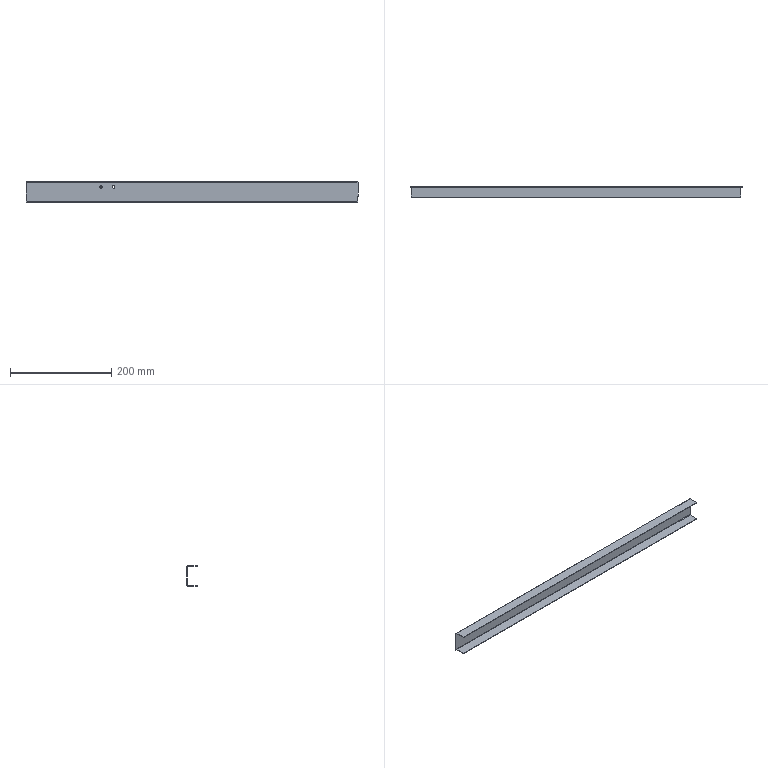Component | SolidWorks | CCQ-1.1-23BendPart-3 | 1 solid | 28 faces | box 655 x 20 x 40 mm | volume 50169 mm3 | plane 20 | cylinder 8 | commonest cylinder face diameters 5 x4 3.473 x2 1.473 x2 | material 304
STEP:
#1=COLOUR_RGB('',0.7922,0.8196,0.9333);
#2=FILL_AREA_STYLE_COLOUR('',#1);
#3=FILL_AREA_STYLE('',(#2));
#4=SURFACE_STYLE_FILL_AREA(#3);
#5=SURFACE_SIDE_STYLE('',(#4));
#6=SURFACE_STYLE_USAGE(.BOTH.,#5);
#7=PRESENTATION_STYLE_ASSIGNMENT((#6));
#8=CARTESIAN_POINT('',(-18.189,-4.114,-3.031));
#9=VERTEX_POINT('',#8);
#10=CARTESIAN_POINT('',(-18.386,-4.114,-3.031));
#11=VERTEX_POINT('',#10);
#12=CARTESIAN_POINT('',(-18.287,-4.114,-3.031));
#13=DIRECTION('',(-0.,1.,0.));
#14=DIRECTION('',(-1.,0.,0.));
#15=AXIS2_PLACEMENT_3D('',#12,#13,#14);
#16=CIRCLE('',#15,0.09843);
#17=EDGE_CURVE('',#9,#11,#16,.T.);
#18=ORIENTED_EDGE('',*,*,#17,.F.);
#19=CARTESIAN_POINT('',(-18.189,-4.075,-3.031));
#20=VERTEX_POINT('',#19);
#21=CARTESIAN_POINT('',(-18.189,-4.469,-3.031));
#22=DIRECTION('',(-0.,1.,0.));
#23=VECTOR('',#22,39.37);
#24=LINE('',#21,#23);
#25=EDGE_CURVE('',#9,#20,#24,.T.);
#26=ORIENTED_EDGE('',*,*,#25,.T.);
#27=CARTESIAN_POINT('',(-18.386,-4.075,-3.031));
#28=VERTEX_POINT('',#27);
#29=CARTESIAN_POINT('',(-18.287,-4.075,-3.031));
#30=DIRECTION('',(-0.,1.,0.));
#31=DIRECTION('',(-1.,0.,0.));
#32=AXIS2_PLACEMENT_3D('',#29,#30,#31);
#33=CIRCLE('',#32,0.09843);
#34=EDGE_CURVE('',#20,#28,#33,.T.);
#35=ORIENTED_EDGE('',*,*,#34,.T.);
#36=CARTESIAN_POINT('',(-18.386,-4.469,-3.031));
#37=DIRECTION('',(-0.,1.,0.));
#38=VECTOR('',#37,39.37);
#39=LINE('',#36,#38);
#40=EDGE_CURVE('',#11,#28,#39,.T.);
#41=ORIENTED_EDGE('',*,*,#40,.F.);
#42=EDGE_LOOP('',(#18,#26,#35,#41));
#43=FACE_OUTER_BOUND('',#42,.T.);
#44=CARTESIAN_POINT('',(-18.287,-4.469,-3.031));
#45=DIRECTION('',(-0.,1.,0.));
#46=DIRECTION('',(-1.,0.,0.));
#47=AXIS2_PLACEMENT_3D('',#44,#45,#46);
#48=CYLINDRICAL_SURFACE('',#47,0.09843);
#49=ADVANCED_FACE('',(#43),#48,.F.);
#50=CARTESIAN_POINT('',(-19.173,-4.114,-3.031));
#51=VERTEX_POINT('',#50);
#52=CARTESIAN_POINT('',(-19.37,-4.114,-3.031));
#53=VERTEX_POINT('',#52);
#54=CARTESIAN_POINT('',(-19.272,-4.114,-3.031));
#55=DIRECTION('',(-0.,1.,0.));
#56=DIRECTION('',(-1.,0.,0.));
#57=AXIS2_PLACEMENT_3D('',#54,#55,#56);
#58=CIRCLE('',#57,0.09843);
#59=EDGE_CURVE('',#51,#53,#58,.T.);
#60=ORIENTED_EDGE('',*,*,#59,.F.);
#61=CARTESIAN_POINT('',(-19.173,-4.075,-3.031));
#62=VERTEX_POINT('',#61);
#63=CARTESIAN_POINT('',(-19.173,-4.469,-3.031));
#64=DIRECTION('',(-0.,1.,0.));
#65=VECTOR('',#64,39.37);
#66=LINE('',#63,#65);
#67=EDGE_CURVE('',#51,#62,#66,.T.);
#68=ORIENTED_EDGE('',*,*,#67,.T.);
#69=CARTESIAN_POINT('',(-19.37,-4.075,-3.031));
#70=VERTEX_POINT('',#69);
#71=CARTESIAN_POINT('',(-19.272,-4.075,-3.031));
#72=DIRECTION('',(-0.,1.,0.));
#73=DIRECTION('',(-1.,0.,0.));
#74=AXIS2_PLACEMENT_3D('',#71,#72,#73);
#75=CIRCLE('',#74,0.09843);
#76=EDGE_CURVE('',#62,#70,#75,.T.);
#77=ORIENTED_EDGE('',*,*,#76,.T.);
#78=CARTESIAN_POINT('',(-19.37,-4.469,-3.031));
#79=DIRECTION('',(-0.,1.,0.));
#80=VECTOR('',#79,39.37);
#81=LINE('',#78,#80);
#82=EDGE_CURVE('',#53,#70,#81,.T.);
#83=ORIENTED_EDGE('',*,*,#82,.F.);
#84=EDGE_LOOP('',(#60,#68,#77,#83));
#85=FACE_OUTER_BOUND('',#84,.T.);
#86=CARTESIAN_POINT('',(-19.272,-4.469,-3.031));
#87=DIRECTION('',(-0.,1.,0.));
#88=DIRECTION('',(-1.,0.,0.));
#89=AXIS2_PLACEMENT_3D('',#86,#87,#88);
#90=CYLINDRICAL_SURFACE('',#89,0.09843);
#91=ADVANCED_FACE('',(#85),#90,.F.);
#92=CARTESIAN_POINT('',(-25.098,-4.114,-3.74));
#93=VERTEX_POINT('',#92);
#94=CARTESIAN_POINT('',(-25.098,-4.075,-3.74));
#95=VERTEX_POINT('',#94);
#96=CARTESIAN_POINT('',(-25.098,-4.143,-3.74));
#97=DIRECTION('',(-0.,1.,0.));
#98=VECTOR('',#97,39.37);
#99=LINE('',#96,#98);
#100=EDGE_CURVE('',#93,#95,#99,.T.);
#101=ORIENTED_EDGE('',*,*,#100,.F.);
#102=CARTESIAN_POINT('',(-25.098,-4.114,-2.706));
#103=VERTEX_POINT('',#102);
#104=CARTESIAN_POINT('',(-25.098,-4.114,-4.213));
#105=DIRECTION('',(-0.,-0.,1.));
#106=VECTOR('',#105,39.37);
#107=LINE('',#104,#106);
#108=EDGE_CURVE('',#93,#103,#107,.T.);
#109=ORIENTED_EDGE('',*,*,#108,.T.);
#110=CARTESIAN_POINT('',(-25.098,-4.075,-2.706));
#111=VERTEX_POINT('',#110);
#112=CARTESIAN_POINT('',(-25.098,-4.114,-2.706));
#113=DIRECTION('',(-0.,1.,0.));
#114=VECTOR('',#113,39.37);
#115=LINE('',#112,#114);
#116=EDGE_CURVE('',#103,#111,#115,.T.);
#117=ORIENTED_EDGE('',*,*,#116,.T.);
#118=CARTESIAN_POINT('',(-25.098,-4.075,-4.213));
#119=DIRECTION('',(-0.,-0.,1.));
#120=VECTOR('',#119,39.37);
#121=LINE('',#118,#120);
#122=EDGE_CURVE('',#95,#111,#121,.T.);
#123=ORIENTED_EDGE('',*,*,#122,.F.);
#124=EDGE_LOOP('',(#101,#109,#117,#123));
#125=FACE_OUTER_BOUND('',#124,.T.);
#126=CARTESIAN_POINT('',(-25.098,-4.143,-4.173));
#127=DIRECTION('',(-1.,-0.,-0.));
#128=DIRECTION('',(-0.,-0.,1.));
#129=AXIS2_PLACEMENT_3D('',#126,#127,#128);
#130=PLANE('',#129);
#131=ADVANCED_FACE('',(#125),#130,.T.);
#132=CARTESIAN_POINT('',(-25.098,-4.114,-2.644));
#133=VERTEX_POINT('',#132);
#134=CARTESIAN_POINT('',(-25.098,-4.114,-2.638));
#135=DIRECTION('',(0.,0.,-1.));
#136=VECTOR('',#135,39.37);
#137=LINE('',#134,#136);
#138=EDGE_CURVE('',#133,#103,#137,.T.);
#139=ORIENTED_EDGE('',*,*,#138,.F.);
#140=CARTESIAN_POINT('',(-25.098,-4.143,-2.706));
#141=DIRECTION('',(1.,0.,0.));
#142=DIRECTION('',(0.,0.,1.));
#143=AXIS2_PLACEMENT_3D('',#140,#141,#142);
#144=CIRCLE('',#143,0.06837);
#145=EDGE_CURVE('',#111,#133,#144,.T.);
#146=ORIENTED_EDGE('',*,*,#145,.F.);
#147=ORIENTED_EDGE('',*,*,#116,.F.);
#148=EDGE_LOOP('',(#139,#146,#147));
#149=FACE_OUTER_BOUND('',#148,.T.);
#150=CARTESIAN_POINT('',(-25.098,-4.143,-2.638));
#151=DIRECTION('',(-1.,-0.,-0.));
#152=DIRECTION('',(-0.,-0.,1.));
#153=AXIS2_PLACEMENT_3D('',#150,#151,#152);
#154=PLANE('',#153);
#155=ADVANCED_FACE('',(#149),#154,.T.);
#156=CARTESIAN_POINT('',(0.689,-4.114,-2.706));
#157=VERTEX_POINT('',#156);
#158=CARTESIAN_POINT('',(0.689,-4.114,-2.644));
#159=VERTEX_POINT('',#158);
#160=CARTESIAN_POINT('',(0.689,-4.114,-2.706));
#161=DIRECTION('',(-0.,-0.,1.));
#162=VECTOR('',#161,39.37);
#163=LINE('',#160,#162);
#164=EDGE_CURVE('',#157,#159,#163,.T.);
#165=ORIENTED_EDGE('',*,*,#164,.F.);
#166=CARTESIAN_POINT('',(0.689,-4.075,-2.706));
#167=VERTEX_POINT('',#166);
#168=CARTESIAN_POINT('',(0.689,-4.075,-2.706));
#169=DIRECTION('',(0.,-1.,-0.));
#170=VECTOR('',#169,39.37);
#171=LINE('',#168,#170);
#172=EDGE_CURVE('',#167,#157,#171,.T.);
#173=ORIENTED_EDGE('',*,*,#172,.F.);
#174=CARTESIAN_POINT('',(0.689,-4.143,-2.706));
#175=DIRECTION('',(1.,0.,0.));
#176=DIRECTION('',(0.,0.,1.));
#177=AXIS2_PLACEMENT_3D('',#174,#175,#176);
#178=CIRCLE('',#177,0.06837);
#179=EDGE_CURVE('',#167,#159,#178,.T.);
#180=ORIENTED_EDGE('',*,*,#179,.T.);
#181=EDGE_LOOP('',(#165,#173,#180));
#182=FACE_OUTER_BOUND('',#181,.T.);
#183=CARTESIAN_POINT('',(0.689,-4.075,-2.706));
#184=DIRECTION('',(1.,0.,0.));
#185=DIRECTION('',(0.,0.,-1.));
#186=AXIS2_PLACEMENT_3D('',#183,#184,#185);
#187=PLANE('',#186);
#188=ADVANCED_FACE('',(#182),#187,.T.);
#189=CARTESIAN_POINT('',(0.689,-4.075,-3.74));
#190=VERTEX_POINT('',#189);
#191=CARTESIAN_POINT('',(0.689,-4.114,-3.74));
#192=VERTEX_POINT('',#191);
#193=CARTESIAN_POINT('',(0.689,-4.143,-3.74));
#194=DIRECTION('',(0.,-1.,-0.));
#195=VECTOR('',#194,39.37);
#196=LINE('',#193,#195);
#197=EDGE_CURVE('',#190,#192,#196,.T.);
#198=ORIENTED_EDGE('',*,*,#197,.F.);
#199=CARTESIAN_POINT('',(0.689,-4.075,-4.213));
#200=DIRECTION('',(-0.,-0.,1.));
#201=VECTOR('',#200,39.37);
#202=LINE('',#199,#201);
#203=EDGE_CURVE('',#190,#167,#202,.T.);
#204=ORIENTED_EDGE('',*,*,#203,.T.);
#205=ORIENTED_EDGE('',*,*,#172,.T.);
#206=CARTESIAN_POINT('',(0.689,-4.114,-4.213));
#207=DIRECTION('',(-0.,-0.,1.));
#208=VECTOR('',#207,39.37);
#209=LINE('',#206,#208);
#210=EDGE_CURVE('',#192,#157,#209,.T.);
#211=ORIENTED_EDGE('',*,*,#210,.F.);
#212=EDGE_LOOP('',(#198,#204,#205,#211));
#213=FACE_OUTER_BOUND('',#212,.T.);
#214=CARTESIAN_POINT('',(0.689,-4.143,-2.677));
#215=DIRECTION('',(1.,0.,0.));
#216=DIRECTION('',(0.,0.,-1.));
#217=AXIS2_PLACEMENT_3D('',#214,#215,#216);
#218=PLANE('',#217);
#219=ADVANCED_FACE('',(#213),#218,.T.);
#220=CARTESIAN_POINT('',(-25.008,-4.862,-2.677));
#221=VERTEX_POINT('',#220);
#222=CARTESIAN_POINT('',(0.5984,-4.862,-2.677));
#223=VERTEX_POINT('',#222);
#224=CARTESIAN_POINT('',(-25.098,-4.862,-2.677));
#225=DIRECTION('',(1.,0.,0.));
#226=VECTOR('',#225,39.37);
#227=LINE('',#224,#226);
#228=EDGE_CURVE('',#221,#223,#227,.T.);
#229=ORIENTED_EDGE('',*,*,#228,.F.);
#230=CARTESIAN_POINT('',(-25.008,-4.143,-2.677));
#231=VERTEX_POINT('',#230);
#232=CARTESIAN_POINT('',(-25.008,-4.075,-2.677));
#233=DIRECTION('',(-0.,1.,0.));
#234=VECTOR('',#233,39.37);
#235=LINE('',#232,#234);
#236=EDGE_CURVE('',#221,#231,#235,.T.);
#237=ORIENTED_EDGE('',*,*,#236,.T.);
#238=CARTESIAN_POINT('',(0.5984,-4.143,-2.677));
#239=VERTEX_POINT('',#238);
#240=CARTESIAN_POINT('',(-25.098,-4.143,-2.677));
#241=DIRECTION('',(1.,0.,0.));
#242=VECTOR('',#241,39.37);
#243=LINE('',#240,#242);
#244=EDGE_CURVE('',#231,#239,#243,.T.);
#245=ORIENTED_EDGE('',*,*,#244,.T.);
#246=CARTESIAN_POINT('',(0.5984,-4.075,-2.677));
#247=DIRECTION('',(0.,-1.,-0.));
#248=VECTOR('',#247,39.37);
#249=LINE('',#246,#248);
#250=EDGE_CURVE('',#239,#223,#249,.T.);
#251=ORIENTED_EDGE('',*,*,#250,.T.);
#252=EDGE_LOOP('',(#229,#237,#245,#251));
#253=FACE_OUTER_BOUND('',#252,.T.);
#254=CARTESIAN_POINT('',(-25.098,-4.075,-2.677));
#255=DIRECTION('',(-0.,-0.,1.));
#256=DIRECTION('',(-0.,1.,0.));
#257=AXIS2_PLACEMENT_3D('',#254,#255,#256);
#258=PLANE('',#257);
#259=ADVANCED_FACE('',(#253),#258,.F.);
#260=CARTESIAN_POINT('',(-25.008,-4.862,-2.638));
#261=VERTEX_POINT('',#260);
#262=CARTESIAN_POINT('',(-25.008,-4.862,-2.638));
#263=DIRECTION('',(-0.,-0.,1.));
#264=VECTOR('',#263,39.37);
#265=LINE('',#262,#264);
#266=EDGE_CURVE('',#221,#261,#265,.T.);
#267=ORIENTED_EDGE('',*,*,#266,.F.);
#268=ORIENTED_EDGE('',*,*,#228,.T.);
#269=CARTESIAN_POINT('',(0.5984,-4.862,-2.638));
#270=VERTEX_POINT('',#269);
#271=CARTESIAN_POINT('',(0.5984,-4.862,-2.638));
#272=DIRECTION('',(0.,0.,-1.));
#273=VECTOR('',#272,39.37);
#274=LINE('',#271,#273);
#275=EDGE_CURVE('',#270,#223,#274,.T.);
#276=ORIENTED_EDGE('',*,*,#275,.F.);
#277=CARTESIAN_POINT('',(-25.098,-4.862,-2.638));
#278=DIRECTION('',(1.,0.,0.));
#279=VECTOR('',#278,39.37);
#280=LINE('',#277,#279);
#281=EDGE_CURVE('',#261,#270,#280,.T.);
#282=ORIENTED_EDGE('',*,*,#281,.F.);
#283=EDGE_LOOP('',(#267,#268,#276,#282));
#284=FACE_OUTER_BOUND('',#283,.T.);
#285=CARTESIAN_POINT('',(-25.098,-4.862,-2.638));
#286=DIRECTION('',(0.,-1.,-0.));
#287=DIRECTION('',(1.,0.,0.));
#288=AXIS2_PLACEMENT_3D('',#285,#286,#287);
#289=PLANE('',#288);
#290=ADVANCED_FACE('',(#284),#289,.T.);
#291=CARTESIAN_POINT('',(-25.008,-4.143,-2.638));
#292=VERTEX_POINT('',#291);
#293=CARTESIAN_POINT('',(-25.008,-4.075,-2.638));
#294=DIRECTION('',(-0.,1.,0.));
#295=VECTOR('',#294,39.37);
#296=LINE('',#293,#295);
#297=EDGE_CURVE('',#261,#292,#296,.T.);
#298=ORIENTED_EDGE('',*,*,#297,.F.);
#299=ORIENTED_EDGE('',*,*,#281,.T.);
#300=CARTESIAN_POINT('',(0.5984,-4.143,-2.638));
#301=VERTEX_POINT('',#300);
#302=CARTESIAN_POINT('',(0.5984,-4.075,-2.638));
#303=DIRECTION('',(0.,-1.,-0.));
#304=VECTOR('',#303,39.37);
#305=LINE('',#302,#304);
#306=EDGE_CURVE('',#301,#270,#305,.T.);
#307=ORIENTED_EDGE('',*,*,#306,.F.);
#308=CARTESIAN_POINT('',(-25.098,-4.143,-2.638));
#309=DIRECTION('',(1.,0.,0.));
#310=VECTOR('',#309,39.37);
#311=LINE('',#308,#310);
#312=EDGE_CURVE('',#292,#301,#311,.T.);
#313=ORIENTED_EDGE('',*,*,#312,.F.);
#314=EDGE_LOOP('',(#298,#299,#307,#313));
#315=FACE_OUTER_BOUND('',#314,.T.);
#316=CARTESIAN_POINT('',(-25.098,-4.075,-2.638));
#317=DIRECTION('',(-0.,-0.,1.));
#318=DIRECTION('',(-0.,1.,0.));
#319=AXIS2_PLACEMENT_3D('',#316,#317,#318);
#320=PLANE('',#319);
#321=ADVANCED_FACE('',(#315),#320,.T.);
#322=CARTESIAN_POINT('',(-25.008,-4.114,-2.644));
#323=VERTEX_POINT('',#322);
#324=CARTESIAN_POINT('',(-25.098,-4.114,-2.644));
#325=DIRECTION('',(-1.,-0.,-0.));
#326=VECTOR('',#325,39.37);
#327=LINE('',#324,#326);
#328=EDGE_CURVE('',#323,#133,#327,.T.);
#329=ORIENTED_EDGE('',*,*,#328,.F.);
#330=CARTESIAN_POINT('',(-25.008,-4.143,-2.706));
#331=DIRECTION('',(-1.,-0.,-0.));
#332=DIRECTION('',(0.,-0.,-1.));
#333=AXIS2_PLACEMENT_3D('',#330,#331,#332);
#334=CIRCLE('',#333,0.06837);
#335=EDGE_CURVE('',#292,#323,#334,.T.);
#336=ORIENTED_EDGE('',*,*,#335,.F.);
#337=ORIENTED_EDGE('',*,*,#312,.T.);
#338=CARTESIAN_POINT('',(0.5984,-4.114,-2.644));
#339=VERTEX_POINT('',#338);
#340=CARTESIAN_POINT('',(0.5984,-4.143,-2.706));
#341=DIRECTION('',(1.,0.,0.));
#342=DIRECTION('',(0.,-0.,1.));
#343=AXIS2_PLACEMENT_3D('',#340,#341,#342);
#344=CIRCLE('',#343,0.06837);
#345=EDGE_CURVE('',#339,#301,#344,.T.);
#346=ORIENTED_EDGE('',*,*,#345,.F.);
#347=CARTESIAN_POINT('',(-25.098,-4.114,-2.644));
#348=DIRECTION('',(-1.,-0.,-0.));
#349=VECTOR('',#348,39.37);
#350=LINE('',#347,#349);
#351=EDGE_CURVE('',#159,#339,#350,.T.);
#352=ORIENTED_EDGE('',*,*,#351,.F.);
#353=ORIENTED_EDGE('',*,*,#179,.F.);
#354=CARTESIAN_POINT('',(-25.098,-4.075,-2.706));
#355=DIRECTION('',(1.,0.,0.));
#356=VECTOR('',#355,39.37);
#357=LINE('',#354,#356);
#358=EDGE_CURVE('',#111,#167,#357,.T.);
#359=ORIENTED_EDGE('',*,*,#358,.F.);
#360=ORIENTED_EDGE('',*,*,#145,.T.);
#361=EDGE_LOOP('',(#329,#336,#337,#346,#352,#353,#359,#360));
#362=FACE_OUTER_BOUND('',#361,.T.);
#363=CARTESIAN_POINT('',(-25.098,-4.143,-2.706));
#364=DIRECTION('',(1.,0.,0.));
#365=DIRECTION('',(0.,0.,-1.));
#366=AXIS2_PLACEMENT_3D('',#363,#364,#365);
#367=CYLINDRICAL_SURFACE('',#366,0.06837);
#368=ADVANCED_FACE('',(#362),#367,.T.);
#369=CARTESIAN_POINT('',(-25.079,-4.075,-3.74));
#370=VERTEX_POINT('',#369);
#371=CARTESIAN_POINT('',(-25.079,-4.075,-4.144));
#372=VERTEX_POINT('',#371);
#373=CARTESIAN_POINT('',(-25.079,-4.075,-4.213));
#374=DIRECTION('',(0.,0.,-1.));
#375=VECTOR('',#374,39.37);
#376=LINE('',#373,#375);
#377=EDGE_CURVE('',#370,#372,#376,.T.);
#378=ORIENTED_EDGE('',*,*,#377,.F.);
#379=CARTESIAN_POINT('',(-25.098,-4.075,-3.74));
#380=DIRECTION('',(1.,0.,0.));
#381=VECTOR('',#380,39.37);
#382=LINE('',#379,#381);
#383=EDGE_CURVE('',#95,#370,#382,.T.);
#384=ORIENTED_EDGE('',*,*,#383,.F.);
#385=ORIENTED_EDGE('',*,*,#122,.T.);
#386=ORIENTED_EDGE('',*,*,#358,.T.);
#387=ORIENTED_EDGE('',*,*,#203,.F.);
#388=CARTESIAN_POINT('',(0.6693,-4.075,-3.74));
#389=VERTEX_POINT('',#388);
#390=CARTESIAN_POINT('',(-25.098,-4.075,-3.74));
#391=DIRECTION('',(1.,0.,0.));
#392=VECTOR('',#391,39.37);
#393=LINE('',#390,#392);
#394=EDGE_CURVE('',#389,#190,#393,.T.);
#395=ORIENTED_EDGE('',*,*,#394,.F.);
#396=CARTESIAN_POINT('',(0.6693,-4.075,-4.144));
#397=VERTEX_POINT('',#396);
#398=CARTESIAN_POINT('',(0.6693,-4.075,-4.213));
#399=DIRECTION('',(-0.,-0.,1.));
#400=VECTOR('',#399,39.37);
#401=LINE('',#398,#400);
#402=EDGE_CURVE('',#397,#389,#401,.T.);
#403=ORIENTED_EDGE('',*,*,#402,.F.);
#404=CARTESIAN_POINT('',(-25.098,-4.075,-4.144));
#405=DIRECTION('',(1.,0.,0.));
#406=VECTOR('',#405,39.37);
#407=LINE('',#404,#406);
#408=EDGE_CURVE('',#372,#397,#407,.T.);
#409=ORIENTED_EDGE('',*,*,#408,.F.);
#410=EDGE_LOOP('',(#378,#384,#385,#386,#387,#395,#403,#409));
#411=FACE_OUTER_BOUND('',#410,.T.);
#412=CARTESIAN_POINT('',(-18.287,-4.075,-3.031));
#413=DIRECTION('',(-0.,1.,0.));
#414=DIRECTION('',(-1.,0.,0.));
#415=AXIS2_PLACEMENT_3D('',#412,#413,#414);
#416=CIRCLE('',#415,0.09843);
#417=EDGE_CURVE('',#28,#20,#416,.T.);
#418=ORIENTED_EDGE('',*,*,#417,.F.);
#419=ORIENTED_EDGE('',*,*,#34,.F.);
#420=EDGE_LOOP('',(#418,#419));
#421=FACE_BOUND('',#420,.T.);
#422=CARTESIAN_POINT('',(-19.272,-4.075,-3.031));
#423=DIRECTION('',(-0.,1.,0.));
#424=DIRECTION('',(-1.,0.,0.));
#425=AXIS2_PLACEMENT_3D('',#422,#423,#424);
#426=CIRCLE('',#425,0.09843);
#427=EDGE_CURVE('',#70,#62,#426,.T.);
#428=ORIENTED_EDGE('',*,*,#427,.F.);
#429=ORIENTED_EDGE('',*,*,#76,.F.);
#430=EDGE_LOOP('',(#428,#429));
#431=FACE_BOUND('',#430,.T.);
#432=CARTESIAN_POINT('',(-25.098,-4.075,-4.213));
#433=DIRECTION('',(-0.,1.,0.));
#434=DIRECTION('',(-1.,-0.,-0.));
#435=AXIS2_PLACEMENT_3D('',#432,#433,#434);
#436=PLANE('',#435);
#437=ADVANCED_FACE('',(#411,#421,#431),#436,.T.);
#438=CARTESIAN_POINT('',(-25.079,-4.114,-4.206));
#439=VERTEX_POINT('',#438);
#440=CARTESIAN_POINT('',(-25.079,-4.143,-4.144));
#441=DIRECTION('',(-1.,-0.,-0.));
#442=DIRECTION('',(0.,-0.,-1.));
#443=AXIS2_PLACEMENT_3D('',#440,#441,#442);
#444=CIRCLE('',#443,0.06837);
#445=EDGE_CURVE('',#372,#439,#444,.T.);
#446=ORIENTED_EDGE('',*,*,#445,.F.);
#447=ORIENTED_EDGE('',*,*,#408,.T.);
#448=CARTESIAN_POINT('',(0.6693,-4.114,-4.206));
#449=VERTEX_POINT('',#448);
#450=CARTESIAN_POINT('',(0.6693,-4.143,-4.144));
#451=DIRECTION('',(1.,0.,0.));
#452=DIRECTION('',(0.,0.,1.));
#453=AXIS2_PLACEMENT_3D('',#450,#451,#452);
#454=CIRCLE('',#453,0.06837);
#455=EDGE_CURVE('',#449,#397,#454,.T.);
#456=ORIENTED_EDGE('',*,*,#455,.F.);
#457=CARTESIAN_POINT('',(0.5984,-4.114,-4.206));
#458=VERTEX_POINT('',#457);
#459=CARTESIAN_POINT('',(-25.098,-4.114,-4.206));
#460=DIRECTION('',(1.,0.,0.));
#461=VECTOR('',#460,39.37);
#462=LINE('',#459,#461);
#463=EDGE_CURVE('',#458,#449,#462,.T.);
#464=ORIENTED_EDGE('',*,*,#463,.F.);
#465=CARTESIAN_POINT('',(0.5984,-4.143,-4.213));
#466=VERTEX_POINT('',#465);
#467=CARTESIAN_POINT('',(0.5984,-4.143,-4.144));
#468=DIRECTION('',(1.,0.,0.));
#469=DIRECTION('',(0.,0.,1.));
#470=AXIS2_PLACEMENT_3D('',#467,#468,#469);
#471=CIRCLE('',#470,0.06837);
#472=EDGE_CURVE('',#466,#458,#471,.T.);
#473=ORIENTED_EDGE('',*,*,#472,.F.);
#474=CARTESIAN_POINT('',(-25.008,-4.143,-4.213));
#475=VERTEX_POINT('',#474);
#476=CARTESIAN_POINT('',(-25.098,-4.143,-4.213));
#477=DIRECTION('',(1.,0.,0.));
#478=VECTOR('',#477,39.37);
#479=LINE('',#476,#478);
#480=EDGE_CURVE('',#475,#466,#479,.T.);
#481=ORIENTED_EDGE('',*,*,#480,.F.);
#482=CARTESIAN_POINT('',(-25.008,-4.114,-4.206));
#483=VERTEX_POINT('',#482);
#484=CARTESIAN_POINT('',(-25.008,-4.143,-4.144));
#485=DIRECTION('',(-1.,-0.,-0.));
#486=DIRECTION('',(0.,0.,-1.));
#487=AXIS2_PLACEMENT_3D('',#484,#485,#486);
#488=CIRCLE('',#487,0.06837);
#489=EDGE_CURVE('',#483,#475,#488,.T.);
#490=ORIENTED_EDGE('',*,*,#489,.F.);
#491=CARTESIAN_POINT('',(-25.098,-4.114,-4.206));
#492=DIRECTION('',(1.,0.,0.));
#493=VECTOR('',#492,39.37);
#494=LINE('',#491,#493);
#495=EDGE_CURVE('',#439,#483,#494,.T.);
#496=ORIENTED_EDGE('',*,*,#495,.F.);
#497=EDGE_LOOP('',(#446,#447,#456,#464,#473,#481,#490,#496));
#498=FACE_OUTER_BOUND('',#497,.T.);
#499=CARTESIAN_POINT('',(-25.098,-4.143,-4.144));
#500=DIRECTION('',(1.,0.,0.));
#501=DIRECTION('',(0.,0.,-1.));
#502=AXIS2_PLACEMENT_3D('',#499,#500,#501);
#503=CYLINDRICAL_SURFACE('',#502,0.06837);
#504=ADVANCED_FACE('',(#498),#503,.T.);
#505=CARTESIAN_POINT('',(-25.008,-4.862,-4.213));
#506=VERTEX_POINT('',#505);
#507=CARTESIAN_POINT('',(-25.008,-4.862,-4.213));
#508=DIRECTION('',(0.,-1.,0.));
#509=VECTOR('',#508,39.37);
#510=LINE('',#507,#509);
#511=EDGE_CURVE('',#475,#506,#510,.T.);
#512=ORIENTED_EDGE('',*,*,#511,.F.);
#513=ORIENTED_EDGE('',*,*,#480,.T.);
#514=CARTESIAN_POINT('',(0.5984,-4.862,-4.213));
#515=VERTEX_POINT('',#514);
#516=CARTESIAN_POINT('',(0.5984,-4.862,-4.213));
#517=DIRECTION('',(-0.,1.,-0.));
#518=VECTOR('',#517,39.37);
#519=LINE('',#516,#518);
#520=EDGE_CURVE('',#515,#466,#519,.T.);
#521=ORIENTED_EDGE('',*,*,#520,.F.);
#522=CARTESIAN_POINT('',(-25.098,-4.862,-4.213));
#523=DIRECTION('',(1.,0.,0.));
#524=VECTOR('',#523,39.37);
#525=LINE('',#522,#524);
#526=EDGE_CURVE('',#506,#515,#525,.T.);
#527=ORIENTED_EDGE('',*,*,#526,.F.);
#528=EDGE_LOOP('',(#512,#513,#521,#527));
#529=FACE_OUTER_BOUND('',#528,.T.);
#530=CARTESIAN_POINT('',(-25.098,-4.862,-4.213));
#531=DIRECTION('',(0.,-0.,-1.));
#532=DIRECTION('',(0.,-1.,0.));
#533=AXIS2_PLACEMENT_3D('',#530,#531,#532);
#534=PLANE('',#533);
#535=ADVANCED_FACE('',(#529),#534,.T.);
#536=CARTESIAN_POINT('',(-25.008,-4.862,-4.173));
#537=VERTEX_POINT('',#536);
#538=CARTESIAN_POINT('',(-25.008,-4.862,-4.173));
#539=DIRECTION('',(-0.,-0.,1.));
#540=VECTOR('',#539,39.37);
#541=LINE('',#538,#540);
#542=EDGE_CURVE('',#506,#537,#541,.T.);
#543=ORIENTED_EDGE('',*,*,#542,.F.);
#544=ORIENTED_EDGE('',*,*,#526,.T.);
#545=CARTESIAN_POINT('',(0.5984,-4.862,-4.173));
#546=VERTEX_POINT('',#545);
#547=CARTESIAN_POINT('',(0.5984,-4.862,-4.173));
#548=DIRECTION('',(0.,0.,-1.));
#549=VECTOR('',#548,39.37);
#550=LINE('',#547,#549);
#551=EDGE_CURVE('',#546,#515,#550,.T.);
#552=ORIENTED_EDGE('',*,*,#551,.F.);
#553=CARTESIAN_POINT('',(-25.098,-4.862,-4.173));
#554=DIRECTION('',(1.,0.,0.));
#555=VECTOR('',#554,39.37);
#556=LINE('',#553,#555);
#557=EDGE_CURVE('',#537,#546,#556,.T.);
#558=ORIENTED_EDGE('',*,*,#557,.F.);
#559=EDGE_LOOP('',(#543,#544,#552,#558));
#560=FACE_OUTER_BOUND('',#559,.T.);
#561=CARTESIAN_POINT('',(-25.098,-4.862,-4.173));
#562=DIRECTION('',(0.,-1.,-0.));
#563=DIRECTION('',(1.,0.,0.));
#564=AXIS2_PLACEMENT_3D('',#561,#562,#563);
#565=PLANE('',#564);
#566=ADVANCED_FACE('',(#560),#565,.T.);
#567=CARTESIAN_POINT('',(-25.008,-4.143,-4.173));
#568=VERTEX_POINT('',#567);
#569=CARTESIAN_POINT('',(0.5984,-4.143,-4.173));
#570=VERTEX_POINT('',#569);
#571=CARTESIAN_POINT('',(-25.098,-4.143,-4.173));
#572=DIRECTION('',(1.,0.,0.));
#573=VECTOR('',#572,39.37);
#574=LINE('',#571,#573);
#575=EDGE_CURVE('',#568,#570,#574,.T.);
#576=ORIENTED_EDGE('',*,*,#575,.F.);
#577=CARTESIAN_POINT('',(-25.008,-4.862,-4.173));
#578=DIRECTION('',(0.,-1.,0.));
#579=VECTOR('',#578,39.37);
#580=LINE('',#577,#579);
#581=EDGE_CURVE('',#568,#537,#580,.T.);
#582=ORIENTED_EDGE('',*,*,#581,.T.);
#583=ORIENTED_EDGE('',*,*,#557,.T.);
#584=CARTESIAN_POINT('',(0.5984,-4.862,-4.173));
#585=DIRECTION('',(-0.,1.,-0.));
#586=VECTOR('',#585,39.37);
#587=LINE('',#584,#586);
#588=EDGE_CURVE('',#546,#570,#587,.T.);
#589=ORIENTED_EDGE('',*,*,#588,.T.);
#590=EDGE_LOOP('',(#576,#582,#583,#589));
#591=FACE_OUTER_BOUND('',#590,.T.);
#592=CARTESIAN_POINT('',(-25.098,-4.862,-4.173));
#593=DIRECTION('',(0.,-0.,-1.));
#594=DIRECTION('',(0.,-1.,0.));
#595=AXIS2_PLACEMENT_3D('',#592,#593,#594);
#596=PLANE('',#595);
#597=ADVANCED_FACE('',(#591),#596,.F.);
#598=CARTESIAN_POINT('',(-25.008,-4.114,-4.144));
#599=VERTEX_POINT('',#598);
#600=CARTESIAN_POINT('',(0.5984,-4.114,-4.144));
#601=VERTEX_POINT('',#600);
#602=CARTESIAN_POINT('',(-25.098,-4.114,-4.144));
#603=DIRECTION('',(1.,0.,0.));
#604=VECTOR('',#603,39.37);
#605=LINE('',#602,#604);
#606=EDGE_CURVE('',#599,#601,#605,.T.);
#607=ORIENTED_EDGE('',*,*,#606,.F.);
#608=CARTESIAN_POINT('',(-25.008,-4.143,-4.144));
#609=DIRECTION('',(-1.,-0.,-0.));
#610=DIRECTION('',(0.,0.,-1.));
#611=AXIS2_PLACEMENT_3D('',#608,#609,#610);
#612=CIRCLE('',#611,0.029);
#613=EDGE_CURVE('',#599,#568,#612,.T.);
#614=ORIENTED_EDGE('',*,*,#613,.T.);
#615=ORIENTED_EDGE('',*,*,#575,.T.);
#616=CARTESIAN_POINT('',(0.5984,-4.143,-4.144));
#617=DIRECTION('',(1.,0.,0.));
#618=DIRECTION('',(0.,0.,1.));
#619=AXIS2_PLACEMENT_3D('',#616,#617,#618);
#620=CIRCLE('',#619,0.029);
#621=EDGE_CURVE('',#570,#601,#620,.T.);
#622=ORIENTED_EDGE('',*,*,#621,.T.);
#623=EDGE_LOOP('',(#607,#614,#615,#622));
#624=FACE_OUTER_BOUND('',#623,.T.);
#625=CARTESIAN_POINT('',(-25.098,-4.143,-4.144));
#626=DIRECTION('',(1.,0.,0.));
#627=DIRECTION('',(0.,0.,-1.));
#628=AXIS2_PLACEMENT_3D('',#625,#626,#627);
#629=CYLINDRICAL_SURFACE('',#628,0.029);
#630=ADVANCED_FACE('',(#624),#629,.F.);
#631=CARTESIAN_POINT('',(-18.287,-4.114,-3.031));
#632=DIRECTION('',(-0.,1.,0.));
#633=DIRECTION('',(-1.,0.,0.));
#634=AXIS2_PLACEMENT_3D('',#631,#632,#633);
#635=CIRCLE('',#634,0.09843);
#636=EDGE_CURVE('',#11,#9,#635,.T.);
#637=ORIENTED_EDGE('',*,*,#636,.T.);
#638=ORIENTED_EDGE('',*,*,#17,.T.);
#639=EDGE_LOOP('',(#637,#638));
#640=FACE_BOUND('',#639,.T.);
#641=CARTESIAN_POINT('',(-19.272,-4.114,-3.031));
#642=DIRECTION('',(-0.,1.,0.));
#643=DIRECTION('',(-1.,0.,0.));
#644=AXIS2_PLACEMENT_3D('',#641,#642,#643);
#645=CIRCLE('',#644,0.09843);
#646=EDGE_CURVE('',#53,#51,#645,.T.);
#647=ORIENTED_EDGE('',*,*,#646,.T.);
#648=ORIENTED_EDGE('',*,*,#59,.T.);
#649=EDGE_LOOP('',(#647,#648));
#650=FACE_BOUND('',#649,.T.);
#651=CARTESIAN_POINT('',(-25.008,-4.114,-2.706));
#652=VERTEX_POINT('',#651);
#653=CARTESIAN_POINT('',(0.5984,-4.114,-2.706));
#654=VERTEX_POINT('',#653);
#655=CARTESIAN_POINT('',(-25.098,-4.114,-2.706));
#656=DIRECTION('',(1.,0.,0.));
#657=VECTOR('',#656,39.37);
#658=LINE('',#655,#657);
#659=EDGE_CURVE('',#652,#654,#658,.T.);
#660=ORIENTED_EDGE('',*,*,#659,.F.);
#661=CARTESIAN_POINT('',(-25.008,-4.114,-3.425));
#662=DIRECTION('',(0.,0.,-1.));
#663=VECTOR('',#662,39.37);
#664=LINE('',#661,#663);
#665=EDGE_CURVE('',#323,#652,#664,.T.);
#666=ORIENTED_EDGE('',*,*,#665,.F.);
#667=ORIENTED_EDGE('',*,*,#328,.T.);
#668=ORIENTED_EDGE('',*,*,#138,.T.);
#669=ORIENTED_EDGE('',*,*,#108,.F.);
#670=CARTESIAN_POINT('',(-25.079,-4.114,-3.74));
#671=VERTEX_POINT('',#670);
#672=CARTESIAN_POINT('',(-25.079,-4.114,-3.74));
#673=DIRECTION('',(-1.,-0.,-0.));
#674=VECTOR('',#673,39.37);
#675=LINE('',#672,#674);
#676=EDGE_CURVE('',#671,#93,#675,.T.);
#677=ORIENTED_EDGE('',*,*,#676,.F.);
#678=CARTESIAN_POINT('',(-25.079,-4.114,-3.978));
#679=DIRECTION('',(-0.,-0.,1.));
#680=VECTOR('',#679,39.37);
#681=LINE('',#678,#680);
#682=EDGE_CURVE('',#439,#671,#681,.T.);
#683=ORIENTED_EDGE('',*,*,#682,.F.);
#684=ORIENTED_EDGE('',*,*,#495,.T.);
#685=CARTESIAN_POINT('',(-25.008,-4.114,-3.425));
#686=DIRECTION('',(0.,0.,-1.));
#687=VECTOR('',#686,39.37);
#688=LINE('',#685,#687);
#689=EDGE_CURVE('',#599,#483,#688,.T.);
#690=ORIENTED_EDGE('',*,*,#689,.F.);
#691=ORIENTED_EDGE('',*,*,#606,.T.);
#692=CARTESIAN_POINT('',(0.5984,-4.114,-3.425));
#693=DIRECTION('',(-0.,-0.,1.));
#694=VECTOR('',#693,39.37);
#695=LINE('',#692,#694);
#696=EDGE_CURVE('',#458,#601,#695,.T.);
#697=ORIENTED_EDGE('',*,*,#696,.F.);
#698=ORIENTED_EDGE('',*,*,#463,.T.);
#699=CARTESIAN_POINT('',(0.6693,-4.114,-3.74));
#700=VERTEX_POINT('',#699);
#701=CARTESIAN_POINT('',(0.6693,-4.114,-3.978));
#702=DIRECTION('',(0.,0.,-1.));
#703=VECTOR('',#702,39.37);
#704=LINE('',#701,#703);
#705=EDGE_CURVE('',#700,#449,#704,.T.);
#706=ORIENTED_EDGE('',*,*,#705,.F.);
#707=CARTESIAN_POINT('',(0.6929,-4.114,-3.74));
#708=DIRECTION('',(-1.,-0.,-0.));
#709=VECTOR('',#708,39.37);
#710=LINE('',#707,#709);
#711=EDGE_CURVE('',#192,#700,#710,.T.);
#712=ORIENTED_EDGE('',*,*,#711,.F.);
#713=ORIENTED_EDGE('',*,*,#210,.T.);
#714=ORIENTED_EDGE('',*,*,#164,.T.);
#715=ORIENTED_EDGE('',*,*,#351,.T.);
#716=CARTESIAN_POINT('',(0.5984,-4.114,-3.425));
#717=DIRECTION('',(-0.,-0.,1.));
#718=VECTOR('',#717,39.37);
#719=LINE('',#716,#718);
#720=EDGE_CURVE('',#654,#339,#719,.T.);
#721=ORIENTED_EDGE('',*,*,#720,.F.);
#722=EDGE_LOOP('',(#660,#666,#667,#668,#669,#677,#683,#684,#690,#691,#697,#698,#706,#712,#713,#714,#715,#721));
#723=FACE_OUTER_BOUND('',#722,.T.);
#724=CARTESIAN_POINT('',(-25.098,-4.114,-4.213));
#725=DIRECTION('',(-0.,1.,0.));
#726=DIRECTION('',(-1.,-0.,-0.));
#727=AXIS2_PLACEMENT_3D('',#724,#725,#726);
#728=PLANE('',#727);
#729=ADVANCED_FACE('',(#640,#650,#723),#728,.F.);
#730=ORIENTED_EDGE('',*,*,#244,.F.);
#731=CARTESIAN_POINT('',(-25.008,-4.143,-2.706));
#732=DIRECTION('',(-1.,-0.,-0.));
#733=DIRECTION('',(0.,0.,-1.));
#734=AXIS2_PLACEMENT_3D('',#731,#732,#733);
#735=CIRCLE('',#734,0.029);
#736=EDGE_CURVE('',#231,#652,#735,.T.);
#737=ORIENTED_EDGE('',*,*,#736,.T.);
#738=ORIENTED_EDGE('',*,*,#659,.T.);
#739=CARTESIAN_POINT('',(0.5984,-4.143,-2.706));
#740=DIRECTION('',(1.,0.,0.));
#741=DIRECTION('',(0.,0.,1.));
#742=AXIS2_PLACEMENT_3D('',#739,#740,#741);
#743=CIRCLE('',#742,0.029);
#744=EDGE_CURVE('',#654,#239,#743,.T.);
#745=ORIENTED_EDGE('',*,*,#744,.T.);
#746=EDGE_LOOP('',(#730,#737,#738,#745));
#747=FACE_OUTER_BOUND('',#746,.T.);
#748=CARTESIAN_POINT('',(-25.098,-4.143,-2.706));
#749=DIRECTION('',(1.,0.,0.));
#750=DIRECTION('',(0.,0.,-1.));
#751=AXIS2_PLACEMENT_3D('',#748,#749,#750);
#752=CYLINDRICAL_SURFACE('',#751,0.029);
#753=ADVANCED_FACE('',(#747),#752,.F.);
#754=ORIENTED_EDGE('',*,*,#67,.F.);
#755=ORIENTED_EDGE('',*,*,#646,.F.);
#756=ORIENTED_EDGE('',*,*,#82,.T.);
#757=ORIENTED_EDGE('',*,*,#427,.T.);
#758=EDGE_LOOP('',(#754,#755,#756,#757));
#759=FACE_OUTER_BOUND('',#758,.T.);
#760=CARTESIAN_POINT('',(-19.272,-4.469,-3.031));
#761=DIRECTION('',(-0.,1.,0.));
#762=DIRECTION('',(-1.,0.,0.));
#763=AXIS2_PLACEMENT_3D('',#760,#761,#762);
#764=CYLINDRICAL_SURFACE('',#763,0.09843);
#765=ADVANCED_FACE('',(#759),#764,.F.);
#766=ORIENTED_EDGE('',*,*,#25,.F.);
#767=ORIENTED_EDGE('',*,*,#636,.F.);
#768=ORIENTED_EDGE('',*,*,#40,.T.);
#769=ORIENTED_EDGE('',*,*,#417,.T.);
#770=EDGE_LOOP('',(#766,#767,#768,#769));
#771=FACE_OUTER_BOUND('',#770,.T.);
#772=CARTESIAN_POINT('',(-18.287,-4.469,-3.031));
#773=DIRECTION('',(-0.,1.,0.));
#774=DIRECTION('',(-1.,0.,0.));
#775=AXIS2_PLACEMENT_3D('',#772,#773,#774);
#776=CYLINDRICAL_SURFACE('',#775,0.09843);
#777=ADVANCED_FACE('',(#771),#776,.F.);
#778=ORIENTED_EDGE('',*,*,#345,.T.);
#779=ORIENTED_EDGE('',*,*,#306,.T.);
#780=ORIENTED_EDGE('',*,*,#275,.T.);
#781=ORIENTED_EDGE('',*,*,#250,.F.);
#782=ORIENTED_EDGE('',*,*,#744,.F.);
#783=ORIENTED_EDGE('',*,*,#720,.T.);
#784=EDGE_LOOP('',(#778,#779,#780,#781,#782,#783));
#785=FACE_OUTER_BOUND('',#784,.T.);
#786=CARTESIAN_POINT('',(0.5984,-4.49,-3.425));
#787=DIRECTION('',(-1.,-0.,-0.));
#788=DIRECTION('',(-0.,-0.,1.));
#789=AXIS2_PLACEMENT_3D('',#786,#787,#788);
#790=PLANE('',#789);
#791=ADVANCED_FACE('',(#785),#790,.F.);
#792=ORIENTED_EDGE('',*,*,#335,.T.);
#793=ORIENTED_EDGE('',*,*,#665,.T.);
#794=ORIENTED_EDGE('',*,*,#736,.F.);
#795=ORIENTED_EDGE('',*,*,#236,.F.);
#796=ORIENTED_EDGE('',*,*,#266,.T.);
#797=ORIENTED_EDGE('',*,*,#297,.T.);
#798=EDGE_LOOP('',(#792,#793,#794,#795,#796,#797));
#799=FACE_OUTER_BOUND('',#798,.T.);
#800=CARTESIAN_POINT('',(-25.008,-4.49,-3.425));
#801=DIRECTION('',(1.,0.,0.));
#802=DIRECTION('',(0.,0.,-1.));
#803=AXIS2_PLACEMENT_3D('',#800,#801,#802);
#804=PLANE('',#803);
#805=ADVANCED_FACE('',(#799),#804,.F.);
#806=ORIENTED_EDGE('',*,*,#472,.T.);
#807=ORIENTED_EDGE('',*,*,#696,.T.);
#808=ORIENTED_EDGE('',*,*,#621,.F.);
#809=ORIENTED_EDGE('',*,*,#588,.F.);
#810=ORIENTED_EDGE('',*,*,#551,.T.);
#811=ORIENTED_EDGE('',*,*,#520,.T.);
#812=EDGE_LOOP('',(#806,#807,#808,#809,#810,#811));
#813=FACE_OUTER_BOUND('',#812,.T.);
#814=CARTESIAN_POINT('',(0.5984,-4.49,-3.425));
#815=DIRECTION('',(-1.,-0.,-0.));
#816=DIRECTION('',(-0.,-0.,1.));
#817=AXIS2_PLACEMENT_3D('',#814,#815,#816);
#818=PLANE('',#817);
#819=ADVANCED_FACE('',(#813),#818,.F.);
#820=ORIENTED_EDGE('',*,*,#402,.T.);
#821=CARTESIAN_POINT('',(0.6693,-4.093,-3.74));
#822=DIRECTION('',(0.,-1.,-0.));
#823=VECTOR('',#822,39.37);
#824=LINE('',#821,#823);
#825=EDGE_CURVE('',#389,#700,#824,.T.);
#826=ORIENTED_EDGE('',*,*,#825,.T.);
#827=ORIENTED_EDGE('',*,*,#705,.T.);
#828=ORIENTED_EDGE('',*,*,#455,.T.);
#829=EDGE_LOOP('',(#820,#826,#827,#828));
#830=FACE_OUTER_BOUND('',#829,.T.);
#831=CARTESIAN_POINT('',(0.6693,-4.093,-3.978));
#832=DIRECTION('',(-1.,-0.,-0.));
#833=DIRECTION('',(-0.,-0.,1.));
#834=AXIS2_PLACEMENT_3D('',#831,#832,#833);
#835=PLANE('',#834);
#836=ADVANCED_FACE('',(#830),#835,.F.);
#837=ORIENTED_EDGE('',*,*,#197,.T.);
#838=ORIENTED_EDGE('',*,*,#711,.T.);
#839=ORIENTED_EDGE('',*,*,#825,.F.);
#840=ORIENTED_EDGE('',*,*,#394,.T.);
#841=EDGE_LOOP('',(#837,#838,#839,#840));
#842=FACE_OUTER_BOUND('',#841,.T.);
#843=CARTESIAN_POINT('',(0.6929,-4.093,-3.74));
#844=DIRECTION('',(-0.,-0.,1.));
#845=DIRECTION('',(1.,0.,0.));
#846=AXIS2_PLACEMENT_3D('',#843,#844,#845);
#847=PLANE('',#846);
#848=ADVANCED_FACE('',(#842),#847,.F.);
#849=ORIENTED_EDGE('',*,*,#489,.T.);
#850=ORIENTED_EDGE('',*,*,#511,.T.);
#851=ORIENTED_EDGE('',*,*,#542,.T.);
#852=ORIENTED_EDGE('',*,*,#581,.F.);
#853=ORIENTED_EDGE('',*,*,#613,.F.);
#854=ORIENTED_EDGE('',*,*,#689,.T.);
#855=EDGE_LOOP('',(#849,#850,#851,#852,#853,#854));
#856=FACE_OUTER_BOUND('',#855,.T.);
#857=CARTESIAN_POINT('',(-25.008,-4.49,-3.425));
#858=DIRECTION('',(1.,0.,0.));
#859=DIRECTION('',(0.,0.,-1.));
#860=AXIS2_PLACEMENT_3D('',#857,#858,#859);
#861=PLANE('',#860);
#862=ADVANCED_FACE('',(#856),#861,.F.);
#863=ORIENTED_EDGE('',*,*,#377,.T.);
#864=ORIENTED_EDGE('',*,*,#445,.T.);
#865=ORIENTED_EDGE('',*,*,#682,.T.);
#866=CARTESIAN_POINT('',(-25.079,-4.093,-3.74));
#867=DIRECTION('',(-0.,1.,0.));
#868=VECTOR('',#867,39.37);
#869=LINE('',#866,#868);
#870=EDGE_CURVE('',#671,#370,#869,.T.);
#871=ORIENTED_EDGE('',*,*,#870,.T.);
#872=EDGE_LOOP('',(#863,#864,#865,#871));
#873=FACE_OUTER_BOUND('',#872,.T.);
#874=CARTESIAN_POINT('',(-25.079,-4.093,-3.978));
#875=DIRECTION('',(1.,0.,0.));
#876=DIRECTION('',(0.,0.,-1.));
#877=AXIS2_PLACEMENT_3D('',#874,#875,#876);
#878=PLANE('',#877);
#879=ADVANCED_FACE('',(#873),#878,.F.);
#880=ORIENTED_EDGE('',*,*,#100,.T.);
#881=ORIENTED_EDGE('',*,*,#383,.T.);
#882=ORIENTED_EDGE('',*,*,#870,.F.);
#883=ORIENTED_EDGE('',*,*,#676,.T.);
#884=EDGE_LOOP('',(#880,#881,#882,#883));
#885=FACE_OUTER_BOUND('',#884,.T.);
#886=CARTESIAN_POINT('',(-25.079,-4.093,-3.74));
#887=DIRECTION('',(-0.,-0.,1.));
#888=DIRECTION('',(1.,0.,0.));
#889=AXIS2_PLACEMENT_3D('',#886,#887,#888);
#890=PLANE('',#889);
#891=ADVANCED_FACE('',(#885),#890,.F.);
#892=CLOSED_SHELL('',(#49,#91,#131,#155,#188,#219,#259,#290,#321,#368,#437,#504,#535,#566,#597,#630,#729,#753,#765,#777,#791,#805,#819,#836,#848,#862,#879,#891));
#893=MANIFOLD_SOLID_BREP('',#892);
#894=STYLED_ITEM('',(#7),#893);
#895=PRESENTATION_LAYER_ASSIGNMENT('','',(#894));
#896=(LENGTH_UNIT()NAMED_UNIT(*)SI_UNIT($,.METRE.));
#897=LENGTH_MEASURE_WITH_UNIT(LENGTH_MEASURE(0.0254),#896);
#898=DIMENSIONAL_EXPONENTS(1.,0.,0.,0.,0.,0.,0.);
#899=(CONVERSION_BASED_UNIT('',#897)LENGTH_UNIT()NAMED_UNIT(#898));
#900=UNCERTAINTY_MEASURE_WITH_UNIT(LENGTH_MEASURE(0.00001),#899,'','');
#901=(NAMED_UNIT(*)PLANE_ANGLE_UNIT()SI_UNIT($,.RADIAN.));
#902=(NAMED_UNIT(*)SI_UNIT($,.STERADIAN.)SOLID_ANGLE_UNIT());
#903=(GEOMETRIC_REPRESENTATION_CONTEXT(3)GLOBAL_UNCERTAINTY_ASSIGNED_CONTEXT((#900))GLOBAL_UNIT_ASSIGNED_CONTEXT((#899,#901,#902))REPRESENTATION_CONTEXT('',''));
#904=MECHANICAL_DESIGN_GEOMETRIC_PRESENTATION_REPRESENTATION('',(#894),#903);
#905=CARTESIAN_POINT('',(0.,0.,0.));
#906=DIRECTION('',(0.,0.,1.));
#907=DIRECTION('',(1.,0.,0.));
#908=AXIS2_PLACEMENT_3D('',#905,#906,#907);
#909=(LENGTH_UNIT()NAMED_UNIT(*)SI_UNIT($,.METRE.));
#910=LENGTH_MEASURE_WITH_UNIT(LENGTH_MEASURE(0.0254),#909);
#911=DIMENSIONAL_EXPONENTS(1.,0.,0.,0.,0.,0.,0.);
#912=(CONVERSION_BASED_UNIT('',#910)LENGTH_UNIT()NAMED_UNIT(#911));
#913=UNCERTAINTY_MEASURE_WITH_UNIT(LENGTH_MEASURE(0.00001),#912,'','');
#914=(NAMED_UNIT(*)PLANE_ANGLE_UNIT()SI_UNIT($,.RADIAN.));
#915=(NAMED_UNIT(*)SI_UNIT($,.STERADIAN.)SOLID_ANGLE_UNIT());
#916=(GEOMETRIC_REPRESENTATION_CONTEXT(3)GLOBAL_UNCERTAINTY_ASSIGNED_CONTEXT((#913))GLOBAL_UNIT_ASSIGNED_CONTEXT((#912,#914,#915))REPRESENTATION_CONTEXT('',''));
#917=ADVANCED_BREP_SHAPE_REPRESENTATION('',(#893,#908),#916);